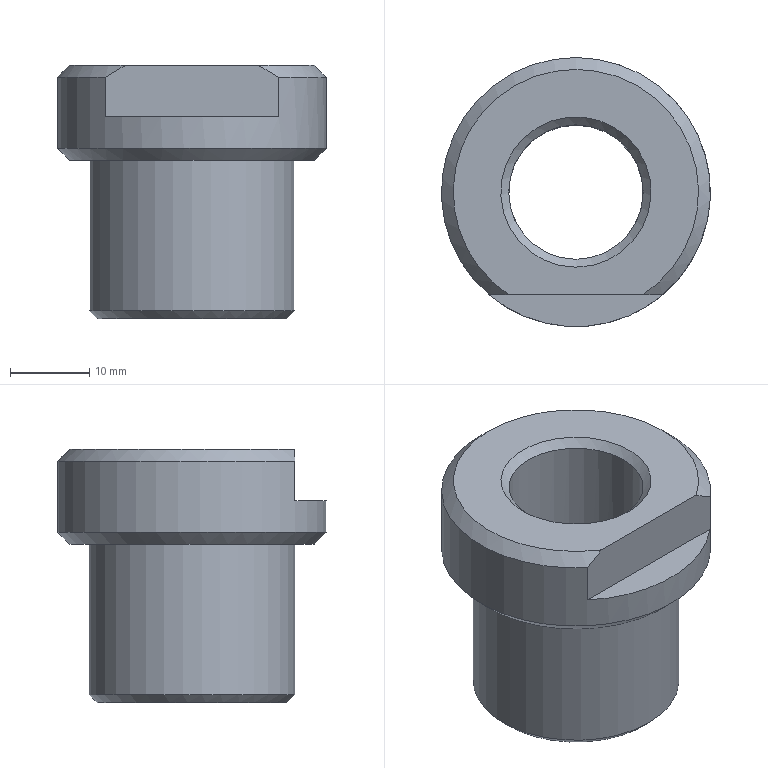Component | NX | DRILL_BUSH_4 | 1 solid | 13 faces | box 34 x 34 x 32 mm | volume 13557 mm3 | plane 5 | cone 5 | cylinder 3 | commonest cylinder face diameters 26 x1 34 x1 17 x1
STEP:
#1=CARTESIAN_POINT('',(0.,0.,0.));
#2=DIRECTION('',(0.,0.,1.));
#3=DIRECTION('',(1.,0.,0.));
#4=AXIS2_PLACEMENT_3D('',#1,#2,#3);
#5=CARTESIAN_POINT('',(62.5,-55.5,100.));
#6=VERTEX_POINT('',#5);
#7=CARTESIAN_POINT('',(62.5,-65.,100.));
#8=DIRECTION('',(0.,0.,1.));
#9=DIRECTION('',(0.,1.,0.));
#10=AXIS2_PLACEMENT_3D('',#7,#8,#9);
#11=CIRCLE('',#10,9.5);
#12=CARTESIAN_POINT('',(62.5,-65.,100.));
#13=DIRECTION('',(0.,0.,-1.));
#14=DIRECTION('',(0.,1.,0.));
#15=AXIS2_PLACEMENT_3D('',#12,#13,#14);
#16=PLANE('',#15);
#17=CARTESIAN_POINT('',(9.5,0.));
#18=CARTESIAN_POINT('',(9.5,-16.454));
#19=CARTESIAN_POINT('',(-4.75,-8.227));
#20=CARTESIAN_POINT('',(-19.,-0.));
#21=CARTESIAN_POINT('',(-4.75,8.227));
#22=CARTESIAN_POINT('',(9.5,16.454));
#23=CARTESIAN_POINT('',(9.5,0.));
#24=(BOUNDED_CURVE()B_SPLINE_CURVE(2,(#17,#18,#19,#20,#21,#22,#23),.UNSPECIFIED.,.T.,.F.)B_SPLINE_CURVE_WITH_KNOTS((1,2,2,2,2,1),(-2.094,0.,2.094,4.189,6.283,8.378),.UNSPECIFIED.)CURVE()GEOMETRIC_REPRESENTATION_ITEM()RATIONAL_B_SPLINE_CURVE((1.,0.5,1.,0.5,1.,0.5,1.))REPRESENTATION_ITEM(''));
#25=(GEOMETRIC_REPRESENTATION_CONTEXT(2)PARAMETRIC_REPRESENTATION_CONTEXT()REPRESENTATION_CONTEXT('',''));
#26=DEFINITIONAL_REPRESENTATION('',(#24),#25);
#27=PCURVE('',#16,#26);
#28=CARTESIAN_POINT('',(62.5,-65.,101.));
#29=DIRECTION('',(0.,0.,-1.));
#30=DIRECTION('',(0.,1.,0.));
#31=AXIS2_PLACEMENT_3D('',#28,#29,#30);
#32=CONICAL_SURFACE('',#31,8.5,0.7854);
#33=CARTESIAN_POINT('',(6.283,1.));
#34=DIRECTION('',(-1.,0.));
#35=VECTOR('',#34,1.);
#36=LINE('',#33,#35);
#37=(GEOMETRIC_REPRESENTATION_CONTEXT(2)PARAMETRIC_REPRESENTATION_CONTEXT()REPRESENTATION_CONTEXT('',''));
#38=DEFINITIONAL_REPRESENTATION('',(#36),#37);
#39=PCURVE('',#32,#38);
#40=SURFACE_CURVE('',#11,(#27,#39),.PCURVE_S1.);
#41=EDGE_CURVE('',#6,#6,#40,.T.);
#42=ORIENTED_EDGE('',*,*,#41,.T.);
#43=EDGE_LOOP('',(#42));
#44=FACE_BOUND('',#43,.T.);
#45=CARTESIAN_POINT('',(62.5,-53.,100.));
#46=VERTEX_POINT('',#45);
#47=CARTESIAN_POINT('',(62.5,-65.,100.));
#48=DIRECTION('',(0.,0.,-1.));
#49=DIRECTION('',(0.,1.,0.));
#50=AXIS2_PLACEMENT_3D('',#47,#48,#49);
#51=CIRCLE('',#50,12.);
#52=CARTESIAN_POINT('',(0.,0.));
#53=DIRECTION('',(1.,0.));
#54=AXIS2_PLACEMENT_2D('',#52,#53);
#55=CIRCLE('',#54,12.);
#56=(GEOMETRIC_REPRESENTATION_CONTEXT(2)PARAMETRIC_REPRESENTATION_CONTEXT()REPRESENTATION_CONTEXT('',''));
#57=DEFINITIONAL_REPRESENTATION('',(#55),#56);
#58=PCURVE('',#16,#57);
#59=CARTESIAN_POINT('',(62.5,-65.,101.));
#60=DIRECTION('',(0.,0.,1.));
#61=DIRECTION('',(0.,-1.,0.));
#62=AXIS2_PLACEMENT_3D('',#59,#60,#61);
#63=CONICAL_SURFACE('',#62,13.,0.7854);
#64=CARTESIAN_POINT('',(9.425,-1.));
#65=DIRECTION('',(-1.,0.));
#66=VECTOR('',#65,1.);
#67=LINE('',#64,#66);
#68=(GEOMETRIC_REPRESENTATION_CONTEXT(2)PARAMETRIC_REPRESENTATION_CONTEXT()REPRESENTATION_CONTEXT('',''));
#69=DEFINITIONAL_REPRESENTATION('',(#67),#68);
#70=PCURVE('',#63,#69);
#71=SURFACE_CURVE('',#51,(#58,#70),.PCURVE_S1.);
#72=EDGE_CURVE('',#46,#46,#71,.T.);
#73=ORIENTED_EDGE('',*,*,#72,.T.);
#74=EDGE_LOOP('',(#73));
#75=FACE_BOUND('',#74,.T.);
#76=ADVANCED_FACE('',(#44,#75),#16,.T.);
#77=CARTESIAN_POINT('',(62.5,-52.,101.));
#78=VERTEX_POINT('',#77);
#79=CARTESIAN_POINT('',(62.5,-65.,101.));
#80=DIRECTION('',(0.,0.,1.));
#81=DIRECTION('',(0.,1.,0.));
#82=AXIS2_PLACEMENT_3D('',#79,#80,#81);
#83=CIRCLE('',#82,13.);
#84=CARTESIAN_POINT('',(62.5,-65.,100.));
#85=DIRECTION('',(0.,0.,1.));
#86=DIRECTION('',(0.,-1.,0.));
#87=AXIS2_PLACEMENT_3D('',#84,#85,#86);
#88=CYLINDRICAL_SURFACE('',#87,13.);
#89=CARTESIAN_POINT('',(3.142,1.));
#90=DIRECTION('',(1.,0.));
#91=VECTOR('',#90,1.);
#92=LINE('',#89,#91);
#93=(GEOMETRIC_REPRESENTATION_CONTEXT(2)PARAMETRIC_REPRESENTATION_CONTEXT()REPRESENTATION_CONTEXT('',''));
#94=DEFINITIONAL_REPRESENTATION('',(#92),#93);
#95=PCURVE('',#88,#94);
#96=CARTESIAN_POINT('',(3.142,0.));
#97=DIRECTION('',(1.,0.));
#98=VECTOR('',#97,1.);
#99=LINE('',#96,#98);
#100=(GEOMETRIC_REPRESENTATION_CONTEXT(2)PARAMETRIC_REPRESENTATION_CONTEXT()REPRESENTATION_CONTEXT('',''));
#101=DEFINITIONAL_REPRESENTATION('',(#99),#100);
#102=PCURVE('',#63,#101);
#103=SURFACE_CURVE('',#83,(#95,#102),.PCURVE_S1.);
#104=EDGE_CURVE('',#78,#78,#103,.T.);
#105=ORIENTED_EDGE('',*,*,#104,.T.);
#106=CARTESIAN_POINT('',(62.5,-52.,120.));
#107=VERTEX_POINT('',#106);
#108=CARTESIAN_POINT('',(62.5,-52.,101.));
#109=CARTESIAN_POINT('',(62.5,-52.,120.));
#110=B_SPLINE_CURVE_WITH_KNOTS('',1,(#108,#109),.UNSPECIFIED.,.F.,.F.,(2,2),(1.,20.),.PIECEWISE_BEZIER_KNOTS.);
#111=CARTESIAN_POINT('',(9.425,0.));
#112=DIRECTION('',(0.,1.));
#113=VECTOR('',#112,1.);
#114=LINE('',#111,#113);
#115=(GEOMETRIC_REPRESENTATION_CONTEXT(2)PARAMETRIC_REPRESENTATION_CONTEXT()REPRESENTATION_CONTEXT('',''));
#116=DEFINITIONAL_REPRESENTATION('',(#114),#115);
#117=PCURVE('',#88,#116);
#118=CARTESIAN_POINT('',(3.142,0.));
#119=DIRECTION('',(0.,1.));
#120=VECTOR('',#119,1.);
#121=LINE('',#118,#120);
#122=(GEOMETRIC_REPRESENTATION_CONTEXT(2)PARAMETRIC_REPRESENTATION_CONTEXT()REPRESENTATION_CONTEXT('',''));
#123=DEFINITIONAL_REPRESENTATION('',(#121),#122);
#124=PCURVE('',#88,#123);
#125=SEAM_CURVE('',#110,(#117,#124),.PCURVE_S1.);
#126=EDGE_CURVE('',#78,#107,#125,.T.);
#127=ORIENTED_EDGE('',*,*,#126,.T.);
#128=CARTESIAN_POINT('',(62.5,-65.,120.));
#129=DIRECTION('',(0.,0.,1.));
#130=DIRECTION('',(0.,1.,0.));
#131=AXIS2_PLACEMENT_3D('',#128,#129,#130);
#132=CIRCLE('',#131,13.);
#133=CARTESIAN_POINT('',(3.142,20.));
#134=DIRECTION('',(1.,0.));
#135=VECTOR('',#134,1.);
#136=LINE('',#133,#135);
#137=(GEOMETRIC_REPRESENTATION_CONTEXT(2)PARAMETRIC_REPRESENTATION_CONTEXT()REPRESENTATION_CONTEXT('',''));
#138=DEFINITIONAL_REPRESENTATION('',(#136),#137);
#139=PCURVE('',#88,#138);
#140=CARTESIAN_POINT('',(62.5,-65.,120.));
#141=DIRECTION('',(0.,0.,-1.));
#142=DIRECTION('',(0.,1.,0.));
#143=AXIS2_PLACEMENT_3D('',#140,#141,#142);
#144=PLANE('',#143);
#145=CARTESIAN_POINT('',(13.,0.));
#146=CARTESIAN_POINT('',(13.,-22.517));
#147=CARTESIAN_POINT('',(-6.5,-11.258));
#148=CARTESIAN_POINT('',(-26.,-0.));
#149=CARTESIAN_POINT('',(-6.5,11.258));
#150=CARTESIAN_POINT('',(13.,22.517));
#151=CARTESIAN_POINT('',(13.,0.));
#152=(BOUNDED_CURVE()B_SPLINE_CURVE(2,(#145,#146,#147,#148,#149,#150,#151),.UNSPECIFIED.,.T.,.F.)B_SPLINE_CURVE_WITH_KNOTS((1,2,2,2,2,1),(-2.094,0.,2.094,4.189,6.283,8.378),.UNSPECIFIED.)CURVE()GEOMETRIC_REPRESENTATION_ITEM()RATIONAL_B_SPLINE_CURVE((1.,0.5,1.,0.5,1.,0.5,1.))REPRESENTATION_ITEM(''));
#153=(GEOMETRIC_REPRESENTATION_CONTEXT(2)PARAMETRIC_REPRESENTATION_CONTEXT()REPRESENTATION_CONTEXT('',''));
#154=DEFINITIONAL_REPRESENTATION('',(#152),#153);
#155=PCURVE('',#144,#154);
#156=SURFACE_CURVE('',#132,(#139,#155),.PCURVE_S1.);
#157=EDGE_CURVE('',#107,#107,#156,.T.);
#158=ORIENTED_EDGE('',*,*,#157,.F.);
#159=ORIENTED_EDGE('',*,*,#126,.F.);
#160=EDGE_LOOP('',(#105,#127,#158,#159));
#161=FACE_BOUND('',#160,.T.);
#162=ADVANCED_FACE('',(#161),#88,.T.);
#163=CARTESIAN_POINT('',(62.5,-74.5,132.));
#164=VERTEX_POINT('',#163);
#165=CARTESIAN_POINT('',(62.5,-65.,132.));
#166=DIRECTION('',(0.,0.,-1.));
#167=DIRECTION('',(0.,-1.,0.));
#168=AXIS2_PLACEMENT_3D('',#165,#166,#167);
#169=CIRCLE('',#168,9.5);
#170=CARTESIAN_POINT('',(62.5,-65.,132.));
#171=DIRECTION('',(0.,0.,1.));
#172=DIRECTION('',(0.,-1.,0.));
#173=AXIS2_PLACEMENT_3D('',#170,#171,#172);
#174=PLANE('',#173);
#175=CARTESIAN_POINT('',(9.5,0.));
#176=CARTESIAN_POINT('',(9.5,-16.454));
#177=CARTESIAN_POINT('',(-4.75,-8.227));
#178=CARTESIAN_POINT('',(-19.,-0.));
#179=CARTESIAN_POINT('',(-4.75,8.227));
#180=CARTESIAN_POINT('',(9.5,16.454));
#181=CARTESIAN_POINT('',(9.5,0.));
#182=(BOUNDED_CURVE()B_SPLINE_CURVE(2,(#175,#176,#177,#178,#179,#180,#181),.UNSPECIFIED.,.T.,.F.)B_SPLINE_CURVE_WITH_KNOTS((1,2,2,2,2,1),(-2.094,0.,2.094,4.189,6.283,8.378),.UNSPECIFIED.)CURVE()GEOMETRIC_REPRESENTATION_ITEM()RATIONAL_B_SPLINE_CURVE((1.,0.5,1.,0.5,1.,0.5,1.))REPRESENTATION_ITEM(''));
#183=(GEOMETRIC_REPRESENTATION_CONTEXT(2)PARAMETRIC_REPRESENTATION_CONTEXT()REPRESENTATION_CONTEXT('',''));
#184=DEFINITIONAL_REPRESENTATION('',(#182),#183);
#185=PCURVE('',#174,#184);
#186=CARTESIAN_POINT('',(62.5,-65.,132.));
#187=DIRECTION('',(0.,0.,1.));
#188=DIRECTION('',(0.,-1.,0.));
#189=AXIS2_PLACEMENT_3D('',#186,#187,#188);
#190=CONICAL_SURFACE('',#189,9.5,0.7854);
#191=CARTESIAN_POINT('',(6.283,0.));
#192=DIRECTION('',(-1.,0.));
#193=VECTOR('',#192,1.);
#194=LINE('',#191,#193);
#195=(GEOMETRIC_REPRESENTATION_CONTEXT(2)PARAMETRIC_REPRESENTATION_CONTEXT()REPRESENTATION_CONTEXT('',''));
#196=DEFINITIONAL_REPRESENTATION('',(#194),#195);
#197=PCURVE('',#190,#196);
#198=SURFACE_CURVE('',#169,(#185,#197),.PCURVE_S1.);
#199=EDGE_CURVE('',#164,#164,#198,.T.);
#200=ORIENTED_EDGE('',*,*,#199,.T.);
#201=EDGE_LOOP('',(#200));
#202=FACE_BOUND('',#201,.T.);
#203=CARTESIAN_POINT('',(70.941,-78.,132.));
#204=VERTEX_POINT('',#203);
#205=CARTESIAN_POINT('',(54.059,-78.,132.));
#206=VERTEX_POINT('',#205);
#207=CARTESIAN_POINT('',(84.5,-78.,132.));
#208=DIRECTION('',(-1.,-0.,0.));
#209=VECTOR('',#208,1.);
#210=LINE('',#207,#209);
#211=CARTESIAN_POINT('',(13.,22.));
#212=DIRECTION('',(0.,-1.));
#213=VECTOR('',#212,1.);
#214=LINE('',#211,#213);
#215=(GEOMETRIC_REPRESENTATION_CONTEXT(2)PARAMETRIC_REPRESENTATION_CONTEXT()REPRESENTATION_CONTEXT('',''));
#216=DEFINITIONAL_REPRESENTATION('',(#214),#215);
#217=PCURVE('',#174,#216);
#218=CARTESIAN_POINT('',(84.5,-78.,125.5));
#219=DIRECTION('',(-0.,1.,0.));
#220=DIRECTION('',(-1.,-0.,0.));
#221=AXIS2_PLACEMENT_3D('',#218,#219,#220);
#222=PLANE('',#221);
#223=CARTESIAN_POINT('',(0.,6.5));
#224=DIRECTION('',(1.,0.));
#225=VECTOR('',#224,1.);
#226=LINE('',#223,#225);
#227=(GEOMETRIC_REPRESENTATION_CONTEXT(2)PARAMETRIC_REPRESENTATION_CONTEXT()REPRESENTATION_CONTEXT('',''));
#228=DEFINITIONAL_REPRESENTATION('',(#226),#227);
#229=PCURVE('',#222,#228);
#230=SURFACE_CURVE('',#210,(#217,#229),.PCURVE_S1.);
#231=EDGE_CURVE('',#204,#206,#230,.T.);
#232=ORIENTED_EDGE('',*,*,#231,.F.);
#233=CARTESIAN_POINT('',(62.5,-65.,132.));
#234=DIRECTION('',(0.,0.,1.));
#235=DIRECTION('',(0.,-1.,0.));
#236=AXIS2_PLACEMENT_3D('',#233,#234,#235);
#237=CIRCLE('',#236,15.5);
#238=CARTESIAN_POINT('',(0.,0.));
#239=DIRECTION('',(1.,0.));
#240=AXIS2_PLACEMENT_2D('',#238,#239);
#241=CIRCLE('',#240,15.5);
#242=(GEOMETRIC_REPRESENTATION_CONTEXT(2)PARAMETRIC_REPRESENTATION_CONTEXT()REPRESENTATION_CONTEXT('',''));
#243=DEFINITIONAL_REPRESENTATION('',(#241),#242);
#244=PCURVE('',#174,#243);
#245=CARTESIAN_POINT('',(62.5,-65.,130.5));
#246=DIRECTION('',(0.,0.,-1.));
#247=DIRECTION('',(0.,1.,0.));
#248=AXIS2_PLACEMENT_3D('',#245,#246,#247);
#249=CONICAL_SURFACE('',#248,17.,0.7854);
#250=CARTESIAN_POINT('',(9.425,-1.5));
#251=DIRECTION('',(-1.,-0.));
#252=VECTOR('',#251,1.);
#253=LINE('',#250,#252);
#254=(GEOMETRIC_REPRESENTATION_CONTEXT(2)PARAMETRIC_REPRESENTATION_CONTEXT()REPRESENTATION_CONTEXT('',''));
#255=DEFINITIONAL_REPRESENTATION('',(#253),#254);
#256=PCURVE('',#249,#255);
#257=SURFACE_CURVE('',#237,(#244,#256),.PCURVE_S1.);
#258=EDGE_CURVE('',#204,#206,#257,.T.);
#259=ORIENTED_EDGE('',*,*,#258,.T.);
#260=EDGE_LOOP('',(#232,#259));
#261=FACE_BOUND('',#260,.T.);
#262=ADVANCED_FACE('',(#202,#261),#174,.T.);
#263=CARTESIAN_POINT('',(62.5,-49.5,120.));
#264=VERTEX_POINT('',#263);
#265=CARTESIAN_POINT('',(62.5,-65.,120.));
#266=DIRECTION('',(0.,0.,-1.));
#267=DIRECTION('',(0.,1.,0.));
#268=AXIS2_PLACEMENT_3D('',#265,#266,#267);
#269=CIRCLE('',#268,15.5);
#270=CARTESIAN_POINT('',(0.,0.));
#271=DIRECTION('',(1.,0.));
#272=AXIS2_PLACEMENT_2D('',#270,#271);
#273=CIRCLE('',#272,15.5);
#274=(GEOMETRIC_REPRESENTATION_CONTEXT(2)PARAMETRIC_REPRESENTATION_CONTEXT()REPRESENTATION_CONTEXT('',''));
#275=DEFINITIONAL_REPRESENTATION('',(#273),#274);
#276=PCURVE('',#144,#275);
#277=CARTESIAN_POINT('',(62.5,-65.,121.5));
#278=DIRECTION('',(0.,0.,1.));
#279=DIRECTION('',(0.,-1.,0.));
#280=AXIS2_PLACEMENT_3D('',#277,#278,#279);
#281=CONICAL_SURFACE('',#280,17.,0.7854);
#282=CARTESIAN_POINT('',(9.425,-1.5));
#283=DIRECTION('',(-1.,0.));
#284=VECTOR('',#283,1.);
#285=LINE('',#282,#284);
#286=(GEOMETRIC_REPRESENTATION_CONTEXT(2)PARAMETRIC_REPRESENTATION_CONTEXT()REPRESENTATION_CONTEXT('',''));
#287=DEFINITIONAL_REPRESENTATION('',(#285),#286);
#288=PCURVE('',#281,#287);
#289=SURFACE_CURVE('',#269,(#276,#288),.PCURVE_S1.);
#290=EDGE_CURVE('',#264,#264,#289,.T.);
#291=ORIENTED_EDGE('',*,*,#290,.T.);
#292=EDGE_LOOP('',(#291));
#293=FACE_BOUND('',#292,.T.);
#294=ORIENTED_EDGE('',*,*,#157,.T.);
#295=EDGE_LOOP('',(#294));
#296=FACE_BOUND('',#295,.T.);
#297=ADVANCED_FACE('',(#293,#296),#144,.T.);
#298=CARTESIAN_POINT('',(62.5,-48.,121.5));
#299=VERTEX_POINT('',#298);
#300=CARTESIAN_POINT('',(51.546,-78.,121.5));
#301=VERTEX_POINT('',#300);
#302=CARTESIAN_POINT('',(62.5,-65.,121.5));
#303=DIRECTION('',(0.,0.,1.));
#304=DIRECTION('',(0.,1.,0.));
#305=AXIS2_PLACEMENT_3D('',#302,#303,#304);
#306=CIRCLE('',#305,17.);
#307=CARTESIAN_POINT('',(62.5,-65.,120.));
#308=DIRECTION('',(0.,0.,1.));
#309=DIRECTION('',(0.,-1.,0.));
#310=AXIS2_PLACEMENT_3D('',#307,#308,#309);
#311=CYLINDRICAL_SURFACE('',#310,17.);
#312=CARTESIAN_POINT('',(9.425,1.5));
#313=DIRECTION('',(1.,0.));
#314=VECTOR('',#313,1.);
#315=LINE('',#312,#314);
#316=(GEOMETRIC_REPRESENTATION_CONTEXT(2)PARAMETRIC_REPRESENTATION_CONTEXT()REPRESENTATION_CONTEXT('',''));
#317=DEFINITIONAL_REPRESENTATION('',(#315),#316);
#318=PCURVE('',#311,#317);
#319=CARTESIAN_POINT('',(3.142,0.));
#320=DIRECTION('',(1.,0.));
#321=VECTOR('',#320,1.);
#322=LINE('',#319,#321);
#323=(GEOMETRIC_REPRESENTATION_CONTEXT(2)PARAMETRIC_REPRESENTATION_CONTEXT()REPRESENTATION_CONTEXT('',''));
#324=DEFINITIONAL_REPRESENTATION('',(#322),#323);
#325=PCURVE('',#281,#324);
#326=SURFACE_CURVE('',#306,(#318,#325),.PCURVE_S1.);
#327=EDGE_CURVE('',#299,#301,#326,.T.);
#328=ORIENTED_EDGE('',*,*,#327,.T.);
#329=CARTESIAN_POINT('',(51.546,-78.,125.5));
#330=VERTEX_POINT('',#329);
#331=CARTESIAN_POINT('',(51.546,-78.,121.5));
#332=CARTESIAN_POINT('',(51.546,-78.,125.5));
#333=B_SPLINE_CURVE_WITH_KNOTS('',1,(#331,#332),.UNSPECIFIED.,.F.,.F.,(2,2),(1.5,5.5),.PIECEWISE_BEZIER_KNOTS.);
#334=CARTESIAN_POINT('',(11.866,0.));
#335=DIRECTION('',(0.,1.));
#336=VECTOR('',#335,1.);
#337=LINE('',#334,#336);
#338=(GEOMETRIC_REPRESENTATION_CONTEXT(2)PARAMETRIC_REPRESENTATION_CONTEXT()REPRESENTATION_CONTEXT('',''));
#339=DEFINITIONAL_REPRESENTATION('',(#337),#338);
#340=PCURVE('',#311,#339);
#341=CARTESIAN_POINT('',(5.583,0.));
#342=DIRECTION('',(0.,1.));
#343=VECTOR('',#342,1.);
#344=LINE('',#341,#343);
#345=(GEOMETRIC_REPRESENTATION_CONTEXT(2)PARAMETRIC_REPRESENTATION_CONTEXT()REPRESENTATION_CONTEXT('',''));
#346=DEFINITIONAL_REPRESENTATION('',(#344),#345);
#347=PCURVE('',#311,#346);
#348=SEAM_CURVE('',#333,(#340,#347),.PCURVE_S1.);
#349=EDGE_CURVE('',#301,#330,#348,.T.);
#350=ORIENTED_EDGE('',*,*,#349,.T.);
#351=CARTESIAN_POINT('',(51.546,-78.,130.5));
#352=VERTEX_POINT('',#351);
#353=CARTESIAN_POINT('',(51.546,-78.,120.));
#354=DIRECTION('',(0.,0.,-1.));
#355=VECTOR('',#354,1.);
#356=LINE('',#353,#355);
#357=CARTESIAN_POINT('',(11.866,0.));
#358=DIRECTION('',(0.,-1.));
#359=VECTOR('',#358,1.);
#360=LINE('',#357,#359);
#361=(GEOMETRIC_REPRESENTATION_CONTEXT(2)PARAMETRIC_REPRESENTATION_CONTEXT()REPRESENTATION_CONTEXT('',''));
#362=DEFINITIONAL_REPRESENTATION('',(#360),#361);
#363=PCURVE('',#311,#362);
#364=CARTESIAN_POINT('',(32.954,-5.5));
#365=DIRECTION('',(0.,-1.));
#366=VECTOR('',#365,1.);
#367=LINE('',#364,#366);
#368=(GEOMETRIC_REPRESENTATION_CONTEXT(2)PARAMETRIC_REPRESENTATION_CONTEXT()REPRESENTATION_CONTEXT('',''));
#369=DEFINITIONAL_REPRESENTATION('',(#367),#368);
#370=PCURVE('',#222,#369);
#371=SURFACE_CURVE('',#356,(#363,#370),.PCURVE_S1.);
#372=EDGE_CURVE('',#352,#330,#371,.T.);
#373=ORIENTED_EDGE('',*,*,#372,.F.);
#374=CARTESIAN_POINT('',(73.454,-78.,130.5));
#375=VERTEX_POINT('',#374);
#376=CARTESIAN_POINT('',(62.5,-65.,130.5));
#377=DIRECTION('',(0.,0.,-1.));
#378=DIRECTION('',(0.,-1.,0.));
#379=AXIS2_PLACEMENT_3D('',#376,#377,#378);
#380=CIRCLE('',#379,17.);
#381=CARTESIAN_POINT('',(12.566,10.5));
#382=DIRECTION('',(-1.,0.));
#383=VECTOR('',#382,1.);
#384=LINE('',#381,#383);
#385=(GEOMETRIC_REPRESENTATION_CONTEXT(2)PARAMETRIC_REPRESENTATION_CONTEXT()REPRESENTATION_CONTEXT('',''));
#386=DEFINITIONAL_REPRESENTATION('',(#384),#385);
#387=PCURVE('',#311,#386);
#388=CARTESIAN_POINT('',(3.142,0.));
#389=DIRECTION('',(1.,-0.));
#390=VECTOR('',#389,1.);
#391=LINE('',#388,#390);
#392=(GEOMETRIC_REPRESENTATION_CONTEXT(2)PARAMETRIC_REPRESENTATION_CONTEXT()REPRESENTATION_CONTEXT('',''));
#393=DEFINITIONAL_REPRESENTATION('',(#391),#392);
#394=PCURVE('',#249,#393);
#395=SURFACE_CURVE('',#380,(#387,#394),.PCURVE_S1.);
#396=EDGE_CURVE('',#352,#375,#395,.T.);
#397=ORIENTED_EDGE('',*,*,#396,.T.);
#398=CARTESIAN_POINT('',(73.454,-78.,125.5));
#399=VERTEX_POINT('',#398);
#400=CARTESIAN_POINT('',(73.454,-78.,120.));
#401=DIRECTION('',(0.,0.,1.));
#402=VECTOR('',#401,1.);
#403=LINE('',#400,#402);
#404=CARTESIAN_POINT('',(6.983,0.));
#405=DIRECTION('',(0.,1.));
#406=VECTOR('',#405,1.);
#407=LINE('',#404,#406);
#408=(GEOMETRIC_REPRESENTATION_CONTEXT(2)PARAMETRIC_REPRESENTATION_CONTEXT()REPRESENTATION_CONTEXT('',''));
#409=DEFINITIONAL_REPRESENTATION('',(#407),#408);
#410=PCURVE('',#311,#409);
#411=CARTESIAN_POINT('',(11.046,-5.5));
#412=DIRECTION('',(0.,1.));
#413=VECTOR('',#412,1.);
#414=LINE('',#411,#413);
#415=(GEOMETRIC_REPRESENTATION_CONTEXT(2)PARAMETRIC_REPRESENTATION_CONTEXT()REPRESENTATION_CONTEXT('',''));
#416=DEFINITIONAL_REPRESENTATION('',(#414),#415);
#417=PCURVE('',#222,#416);
#418=SURFACE_CURVE('',#403,(#410,#417),.PCURVE_S1.);
#419=EDGE_CURVE('',#399,#375,#418,.T.);
#420=ORIENTED_EDGE('',*,*,#419,.F.);
#421=CARTESIAN_POINT('',(62.5,-65.,125.5));
#422=DIRECTION('',(0.,0.,-1.));
#423=DIRECTION('',(0.,-1.,0.));
#424=AXIS2_PLACEMENT_3D('',#421,#422,#423);
#425=CIRCLE('',#424,17.);
#426=CARTESIAN_POINT('',(12.566,5.5));
#427=DIRECTION('',(-1.,0.));
#428=VECTOR('',#427,1.);
#429=LINE('',#426,#428);
#430=(GEOMETRIC_REPRESENTATION_CONTEXT(2)PARAMETRIC_REPRESENTATION_CONTEXT()REPRESENTATION_CONTEXT('',''));
#431=DEFINITIONAL_REPRESENTATION('',(#429),#430);
#432=PCURVE('',#311,#431);
#433=CARTESIAN_POINT('',(62.5,-65.,125.5));
#434=DIRECTION('',(0.,0.,1.));
#435=DIRECTION('',(0.,-1.,0.));
#436=AXIS2_PLACEMENT_3D('',#433,#434,#435);
#437=PLANE('',#436);
#438=CARTESIAN_POINT('',(17.,0.));
#439=CARTESIAN_POINT('',(17.,-29.445));
#440=CARTESIAN_POINT('',(-8.5,-14.722));
#441=CARTESIAN_POINT('',(-34.,-0.));
#442=CARTESIAN_POINT('',(-8.5,14.722));
#443=CARTESIAN_POINT('',(17.,29.445));
#444=CARTESIAN_POINT('',(17.,0.));
#445=(BOUNDED_CURVE()B_SPLINE_CURVE(2,(#438,#439,#440,#441,#442,#443,#444),.UNSPECIFIED.,.T.,.F.)B_SPLINE_CURVE_WITH_KNOTS((1,2,2,2,2,1),(-2.094,0.,2.094,4.189,6.283,8.378),.UNSPECIFIED.)CURVE()GEOMETRIC_REPRESENTATION_ITEM()RATIONAL_B_SPLINE_CURVE((1.,0.5,1.,0.5,1.,0.5,1.))REPRESENTATION_ITEM(''));
#446=(GEOMETRIC_REPRESENTATION_CONTEXT(2)PARAMETRIC_REPRESENTATION_CONTEXT()REPRESENTATION_CONTEXT('',''));
#447=DEFINITIONAL_REPRESENTATION('',(#445),#446);
#448=PCURVE('',#437,#447);
#449=SURFACE_CURVE('',#425,(#432,#448),.PCURVE_S1.);
#450=EDGE_CURVE('',#399,#330,#449,.T.);
#451=ORIENTED_EDGE('',*,*,#450,.T.);
#452=ORIENTED_EDGE('',*,*,#349,.F.);
#453=CARTESIAN_POINT('',(62.5,-65.,121.5));
#454=DIRECTION('',(0.,0.,1.));
#455=DIRECTION('',(0.,1.,0.));
#456=AXIS2_PLACEMENT_3D('',#453,#454,#455);
#457=CIRCLE('',#456,17.);
#458=CARTESIAN_POINT('',(3.142,1.5));
#459=DIRECTION('',(1.,0.));
#460=VECTOR('',#459,1.);
#461=LINE('',#458,#460);
#462=(GEOMETRIC_REPRESENTATION_CONTEXT(2)PARAMETRIC_REPRESENTATION_CONTEXT()REPRESENTATION_CONTEXT('',''));
#463=DEFINITIONAL_REPRESENTATION('',(#461),#462);
#464=PCURVE('',#311,#463);
#465=CARTESIAN_POINT('',(3.142,0.));
#466=DIRECTION('',(1.,-0.));
#467=VECTOR('',#466,1.);
#468=LINE('',#465,#467);
#469=(GEOMETRIC_REPRESENTATION_CONTEXT(2)PARAMETRIC_REPRESENTATION_CONTEXT()REPRESENTATION_CONTEXT('',''));
#470=DEFINITIONAL_REPRESENTATION('',(#468),#469);
#471=PCURVE('',#281,#470);
#472=SURFACE_CURVE('',#457,(#464,#471),.PCURVE_S1.);
#473=EDGE_CURVE('',#301,#299,#472,.T.);
#474=ORIENTED_EDGE('',*,*,#473,.T.);
#475=EDGE_LOOP('',(#328,#350,#373,#397,#420,#451,#452,#474));
#476=FACE_BOUND('',#475,.T.);
#477=ADVANCED_FACE('',(#476),#311,.T.);
#478=CARTESIAN_POINT('',(62.5,-56.5,101.));
#479=VERTEX_POINT('',#478);
#480=CARTESIAN_POINT('',(62.5,-65.,101.));
#481=DIRECTION('',(0.,0.,-1.));
#482=DIRECTION('',(0.,1.,0.));
#483=AXIS2_PLACEMENT_3D('',#480,#481,#482);
#484=CIRCLE('',#483,8.5);
#485=CARTESIAN_POINT('',(62.5,-65.,132.));
#486=DIRECTION('',(0.,0.,-1.));
#487=DIRECTION('',(0.,1.,0.));
#488=AXIS2_PLACEMENT_3D('',#485,#486,#487);
#489=CYLINDRICAL_SURFACE('',#488,8.5);
#490=CARTESIAN_POINT('',(0.,31.));
#491=DIRECTION('',(1.,0.));
#492=VECTOR('',#491,1.);
#493=LINE('',#490,#492);
#494=(GEOMETRIC_REPRESENTATION_CONTEXT(2)PARAMETRIC_REPRESENTATION_CONTEXT()REPRESENTATION_CONTEXT('',''));
#495=DEFINITIONAL_REPRESENTATION('',(#493),#494);
#496=PCURVE('',#489,#495);
#497=CARTESIAN_POINT('',(0.,0.));
#498=DIRECTION('',(1.,0.));
#499=VECTOR('',#498,1.);
#500=LINE('',#497,#499);
#501=(GEOMETRIC_REPRESENTATION_CONTEXT(2)PARAMETRIC_REPRESENTATION_CONTEXT()REPRESENTATION_CONTEXT('',''));
#502=DEFINITIONAL_REPRESENTATION('',(#500),#501);
#503=PCURVE('',#32,#502);
#504=SURFACE_CURVE('',#484,(#496,#503),.PCURVE_S1.);
#505=EDGE_CURVE('',#479,#479,#504,.T.);
#506=ORIENTED_EDGE('',*,*,#505,.F.);
#507=CARTESIAN_POINT('',(62.5,-56.5,131.));
#508=VERTEX_POINT('',#507);
#509=CARTESIAN_POINT('',(62.5,-56.5,131.));
#510=CARTESIAN_POINT('',(62.5,-56.5,101.));
#511=B_SPLINE_CURVE_WITH_KNOTS('',1,(#509,#510),.UNSPECIFIED.,.F.,.F.,(2,2),(1.,31.),.PIECEWISE_BEZIER_KNOTS.);
#512=CARTESIAN_POINT('',(0.,0.));
#513=DIRECTION('',(0.,1.));
#514=VECTOR('',#513,1.);
#515=LINE('',#512,#514);
#516=(GEOMETRIC_REPRESENTATION_CONTEXT(2)PARAMETRIC_REPRESENTATION_CONTEXT()REPRESENTATION_CONTEXT('',''));
#517=DEFINITIONAL_REPRESENTATION('',(#515),#516);
#518=PCURVE('',#489,#517);
#519=CARTESIAN_POINT('',(6.283,0.));
#520=DIRECTION('',(0.,1.));
#521=VECTOR('',#520,1.);
#522=LINE('',#519,#521);
#523=(GEOMETRIC_REPRESENTATION_CONTEXT(2)PARAMETRIC_REPRESENTATION_CONTEXT()REPRESENTATION_CONTEXT('',''));
#524=DEFINITIONAL_REPRESENTATION('',(#522),#523);
#525=PCURVE('',#489,#524);
#526=SEAM_CURVE('',#511,(#518,#525),.PCURVE_S1.);
#527=EDGE_CURVE('',#508,#479,#526,.T.);
#528=ORIENTED_EDGE('',*,*,#527,.F.);
#529=CARTESIAN_POINT('',(62.5,-73.5,131.));
#530=VERTEX_POINT('',#529);
#531=CARTESIAN_POINT('',(62.5,-65.,131.));
#532=DIRECTION('',(0.,0.,1.));
#533=DIRECTION('',(0.,-1.,0.));
#534=AXIS2_PLACEMENT_3D('',#531,#532,#533);
#535=CIRCLE('',#534,8.5);
#536=CARTESIAN_POINT('',(3.142,1.));
#537=DIRECTION('',(-1.,0.));
#538=VECTOR('',#537,1.);
#539=LINE('',#536,#538);
#540=(GEOMETRIC_REPRESENTATION_CONTEXT(2)PARAMETRIC_REPRESENTATION_CONTEXT()REPRESENTATION_CONTEXT('',''));
#541=DEFINITIONAL_REPRESENTATION('',(#539),#540);
#542=PCURVE('',#489,#541);
#543=CARTESIAN_POINT('',(0.,-1.));
#544=DIRECTION('',(1.,0.));
#545=VECTOR('',#544,1.);
#546=LINE('',#543,#545);
#547=(GEOMETRIC_REPRESENTATION_CONTEXT(2)PARAMETRIC_REPRESENTATION_CONTEXT()REPRESENTATION_CONTEXT('',''));
#548=DEFINITIONAL_REPRESENTATION('',(#546),#547);
#549=PCURVE('',#190,#548);
#550=SURFACE_CURVE('',#535,(#542,#549),.PCURVE_S1.);
#551=EDGE_CURVE('',#530,#508,#550,.T.);
#552=ORIENTED_EDGE('',*,*,#551,.F.);
#553=CARTESIAN_POINT('',(62.5,-65.,131.));
#554=DIRECTION('',(0.,0.,1.));
#555=DIRECTION('',(0.,-1.,0.));
#556=AXIS2_PLACEMENT_3D('',#553,#554,#555);
#557=CIRCLE('',#556,8.5);
#558=CARTESIAN_POINT('',(9.425,1.));
#559=DIRECTION('',(-1.,0.));
#560=VECTOR('',#559,1.);
#561=LINE('',#558,#560);
#562=(GEOMETRIC_REPRESENTATION_CONTEXT(2)PARAMETRIC_REPRESENTATION_CONTEXT()REPRESENTATION_CONTEXT('',''));
#563=DEFINITIONAL_REPRESENTATION('',(#561),#562);
#564=PCURVE('',#489,#563);
#565=CARTESIAN_POINT('',(0.,-1.));
#566=DIRECTION('',(1.,0.));
#567=VECTOR('',#566,1.);
#568=LINE('',#565,#567);
#569=(GEOMETRIC_REPRESENTATION_CONTEXT(2)PARAMETRIC_REPRESENTATION_CONTEXT()REPRESENTATION_CONTEXT('',''));
#570=DEFINITIONAL_REPRESENTATION('',(#568),#569);
#571=PCURVE('',#190,#570);
#572=SURFACE_CURVE('',#557,(#564,#571),.PCURVE_S1.);
#573=EDGE_CURVE('',#508,#530,#572,.T.);
#574=ORIENTED_EDGE('',*,*,#573,.F.);
#575=ORIENTED_EDGE('',*,*,#527,.T.);
#576=EDGE_LOOP('',(#506,#528,#552,#574,#575));
#577=FACE_BOUND('',#576,.F.);
#578=ADVANCED_FACE('',(#577),#489,.F.);
#579=ORIENTED_EDGE('',*,*,#419,.T.);
#580=CARTESIAN_POINT('',(73.454,-78.,130.5));
#581=CARTESIAN_POINT('',(72.634,-78.,131.028));
#582=CARTESIAN_POINT('',(71.798,-78.,131.533));
#583=CARTESIAN_POINT('',(70.941,-78.,132.));
#584=B_SPLINE_CURVE_WITH_KNOTS('',3,(#580,#581,#582,#583),.UNSPECIFIED.,.F.,.F.,(4,4),(0.,1.),.PIECEWISE_BEZIER_KNOTS.);
#585=CARTESIAN_POINT('',(11.046,5.));
#586=CARTESIAN_POINT('',(11.866,5.528));
#587=CARTESIAN_POINT('',(12.702,6.033));
#588=CARTESIAN_POINT('',(13.559,6.5));
#589=B_SPLINE_CURVE_WITH_KNOTS('',3,(#585,#586,#587,#588),.UNSPECIFIED.,.F.,.F.,(4,4),(0.,1.),.PIECEWISE_BEZIER_KNOTS.);
#590=(GEOMETRIC_REPRESENTATION_CONTEXT(2)PARAMETRIC_REPRESENTATION_CONTEXT()REPRESENTATION_CONTEXT('',''));
#591=DEFINITIONAL_REPRESENTATION('',(#589),#590);
#592=PCURVE('',#222,#591);
#593=CARTESIAN_POINT('',(8.725,0.));
#594=CARTESIAN_POINT('',(8.726,-0.02402));
#595=CARTESIAN_POINT('',(8.73,-0.07197));
#596=CARTESIAN_POINT('',(8.735,-0.1436));
#597=CARTESIAN_POINT('',(8.74,-0.2149));
#598=CARTESIAN_POINT('',(8.745,-0.2859));
#599=CARTESIAN_POINT('',(8.75,-0.3565));
#600=CARTESIAN_POINT('',(8.756,-0.4269));
#601=CARTESIAN_POINT('',(8.761,-0.4968));
#602=CARTESIAN_POINT('',(8.767,-0.5665));
#603=CARTESIAN_POINT('',(8.772,-0.6358));
#604=CARTESIAN_POINT('',(8.778,-0.7047));
#605=CARTESIAN_POINT('',(8.783,-0.7732));
#606=CARTESIAN_POINT('',(8.789,-0.8414));
#607=CARTESIAN_POINT('',(8.795,-0.9091));
#608=CARTESIAN_POINT('',(8.8,-0.9765));
#609=CARTESIAN_POINT('',(8.806,-1.043));
#610=CARTESIAN_POINT('',(8.812,-1.11));
#611=CARTESIAN_POINT('',(8.818,-1.176));
#612=CARTESIAN_POINT('',(8.824,-1.242));
#613=CARTESIAN_POINT('',(8.83,-1.307));
#614=CARTESIAN_POINT('',(8.836,-1.372));
#615=CARTESIAN_POINT('',(8.843,-1.436));
#616=CARTESIAN_POINT('',(8.847,-1.479));
#617=CARTESIAN_POINT('',(8.849,-1.5));
#618=B_SPLINE_CURVE_WITH_KNOTS('',3,(#593,#594,#595,#596,#597,#598,#599,#600,#601,#602,#603,#604,#605,#606,#607,#608,#609,#610,#611,#612,#613,#614,#615,#616,#617),.UNSPECIFIED.,.F.,.F.,(4,1,1,1,1,1,1,1,1,1,1,1,1,1,1,1,1,1,1,1,1,1,4),(0.,0.04545,0.09091,0.1364,0.1818,0.2273,0.2727,0.3182,0.3636,0.4091,0.4545,0.5,0.5455,0.5909,0.6364,0.6818,0.7273,0.7727,0.8182,0.8636,0.9091,0.9545,1.),.QUASI_UNIFORM_KNOTS.);
#619=(GEOMETRIC_REPRESENTATION_CONTEXT(2)PARAMETRIC_REPRESENTATION_CONTEXT()REPRESENTATION_CONTEXT('',''));
#620=DEFINITIONAL_REPRESENTATION('',(#618),#619);
#621=PCURVE('',#249,#620);
#622=SURFACE_CURVE('',#584,(#592,#621),.PCURVE_S1.);
#623=EDGE_CURVE('',#375,#204,#622,.T.);
#624=ORIENTED_EDGE('',*,*,#623,.T.);
#625=ORIENTED_EDGE('',*,*,#231,.T.);
#626=CARTESIAN_POINT('',(54.059,-78.,132.));
#627=CARTESIAN_POINT('',(53.202,-78.,131.533));
#628=CARTESIAN_POINT('',(52.366,-78.,131.028));
#629=CARTESIAN_POINT('',(51.546,-78.,130.5));
#630=B_SPLINE_CURVE_WITH_KNOTS('',3,(#626,#627,#628,#629),.UNSPECIFIED.,.F.,.F.,(4,4),(0.,1.),.PIECEWISE_BEZIER_KNOTS.);
#631=CARTESIAN_POINT('',(30.441,6.5));
#632=CARTESIAN_POINT('',(31.298,6.033));
#633=CARTESIAN_POINT('',(32.134,5.528));
#634=CARTESIAN_POINT('',(32.954,5.));
#635=B_SPLINE_CURVE_WITH_KNOTS('',3,(#631,#632,#633,#634),.UNSPECIFIED.,.F.,.F.,(4,4),(0.,1.),.PIECEWISE_BEZIER_KNOTS.);
#636=(GEOMETRIC_REPRESENTATION_CONTEXT(2)PARAMETRIC_REPRESENTATION_CONTEXT()REPRESENTATION_CONTEXT('',''));
#637=DEFINITIONAL_REPRESENTATION('',(#635),#636);
#638=PCURVE('',#222,#637);
#639=CARTESIAN_POINT('',(3.717,-1.5));
#640=CARTESIAN_POINT('',(3.72,-1.479));
#641=CARTESIAN_POINT('',(3.724,-1.436));
#642=CARTESIAN_POINT('',(3.73,-1.372));
#643=CARTESIAN_POINT('',(3.736,-1.307));
#644=CARTESIAN_POINT('',(3.742,-1.242));
#645=CARTESIAN_POINT('',(3.748,-1.176));
#646=CARTESIAN_POINT('',(3.754,-1.11));
#647=CARTESIAN_POINT('',(3.76,-1.043));
#648=CARTESIAN_POINT('',(3.766,-0.9765));
#649=CARTESIAN_POINT('',(3.772,-0.9091));
#650=CARTESIAN_POINT('',(3.778,-0.8414));
#651=CARTESIAN_POINT('',(3.783,-0.7732));
#652=CARTESIAN_POINT('',(3.789,-0.7047));
#653=CARTESIAN_POINT('',(3.794,-0.6358));
#654=CARTESIAN_POINT('',(3.8,-0.5665));
#655=CARTESIAN_POINT('',(3.805,-0.4968));
#656=CARTESIAN_POINT('',(3.811,-0.4269));
#657=CARTESIAN_POINT('',(3.816,-0.3565));
#658=CARTESIAN_POINT('',(3.821,-0.2859));
#659=CARTESIAN_POINT('',(3.826,-0.2149));
#660=CARTESIAN_POINT('',(3.832,-0.1436));
#661=CARTESIAN_POINT('',(3.837,-0.07197));
#662=CARTESIAN_POINT('',(3.84,-0.02402));
#663=CARTESIAN_POINT('',(3.842,-0.));
#664=B_SPLINE_CURVE_WITH_KNOTS('',3,(#639,#640,#641,#642,#643,#644,#645,#646,#647,#648,#649,#650,#651,#652,#653,#654,#655,#656,#657,#658,#659,#660,#661,#662,#663),.UNSPECIFIED.,.F.,.F.,(4,1,1,1,1,1,1,1,1,1,1,1,1,1,1,1,1,1,1,1,1,1,4),(0.,0.04545,0.09091,0.1364,0.1818,0.2273,0.2727,0.3182,0.3636,0.4091,0.4545,0.5,0.5455,0.5909,0.6364,0.6818,0.7273,0.7727,0.8182,0.8636,0.9091,0.9545,1.),.QUASI_UNIFORM_KNOTS.);
#665=(GEOMETRIC_REPRESENTATION_CONTEXT(2)PARAMETRIC_REPRESENTATION_CONTEXT()REPRESENTATION_CONTEXT('',''));
#666=DEFINITIONAL_REPRESENTATION('',(#664),#665);
#667=PCURVE('',#249,#666);
#668=SURFACE_CURVE('',#630,(#638,#667),.PCURVE_S1.);
#669=EDGE_CURVE('',#206,#352,#668,.T.);
#670=ORIENTED_EDGE('',*,*,#669,.T.);
#671=ORIENTED_EDGE('',*,*,#372,.T.);
#672=CARTESIAN_POINT('',(84.5,-78.,125.5));
#673=DIRECTION('',(1.,0.,0.));
#674=VECTOR('',#673,1.);
#675=LINE('',#672,#674);
#676=CARTESIAN_POINT('',(0.,0.));
#677=DIRECTION('',(-1.,0.));
#678=VECTOR('',#677,1.);
#679=LINE('',#676,#678);
#680=(GEOMETRIC_REPRESENTATION_CONTEXT(2)PARAMETRIC_REPRESENTATION_CONTEXT()REPRESENTATION_CONTEXT('',''));
#681=DEFINITIONAL_REPRESENTATION('',(#679),#680);
#682=PCURVE('',#222,#681);
#683=CARTESIAN_POINT('',(13.,22.));
#684=DIRECTION('',(-0.,1.));
#685=VECTOR('',#684,1.);
#686=LINE('',#683,#685);
#687=(GEOMETRIC_REPRESENTATION_CONTEXT(2)PARAMETRIC_REPRESENTATION_CONTEXT()REPRESENTATION_CONTEXT('',''));
#688=DEFINITIONAL_REPRESENTATION('',(#686),#687);
#689=PCURVE('',#437,#688);
#690=SURFACE_CURVE('',#675,(#682,#689),.PCURVE_S1.);
#691=EDGE_CURVE('',#330,#399,#690,.T.);
#692=ORIENTED_EDGE('',*,*,#691,.T.);
#693=EDGE_LOOP('',(#579,#624,#625,#670,#671,#692));
#694=FACE_BOUND('',#693,.T.);
#695=ADVANCED_FACE('',(#694),#222,.F.);
#696=ORIENTED_EDGE('',*,*,#691,.F.);
#697=ORIENTED_EDGE('',*,*,#450,.F.);
#698=EDGE_LOOP('',(#696,#697));
#699=FACE_BOUND('',#698,.T.);
#700=ADVANCED_FACE('',(#699),#437,.T.);
#701=ORIENTED_EDGE('',*,*,#290,.F.);
#702=CARTESIAN_POINT('',(62.5,-49.5,120.));
#703=CARTESIAN_POINT('',(62.5,-48.,121.5));
#704=B_SPLINE_CURVE_WITH_KNOTS('',1,(#702,#703),.UNSPECIFIED.,.F.,.F.,(2,2),(-2.121,0.),.PIECEWISE_BEZIER_KNOTS.);
#705=CARTESIAN_POINT('',(9.425,0.));
#706=DIRECTION('',(0.,1.));
#707=VECTOR('',#706,1.);
#708=LINE('',#705,#707);
#709=(GEOMETRIC_REPRESENTATION_CONTEXT(2)PARAMETRIC_REPRESENTATION_CONTEXT()REPRESENTATION_CONTEXT('',''));
#710=DEFINITIONAL_REPRESENTATION('',(#708),#709);
#711=PCURVE('',#281,#710);
#712=CARTESIAN_POINT('',(3.142,0.));
#713=DIRECTION('',(0.,1.));
#714=VECTOR('',#713,1.);
#715=LINE('',#712,#714);
#716=(GEOMETRIC_REPRESENTATION_CONTEXT(2)PARAMETRIC_REPRESENTATION_CONTEXT()REPRESENTATION_CONTEXT('',''));
#717=DEFINITIONAL_REPRESENTATION('',(#715),#716);
#718=PCURVE('',#281,#717);
#719=SEAM_CURVE('',#704,(#711,#718),.PCURVE_S1.);
#720=EDGE_CURVE('',#264,#299,#719,.T.);
#721=ORIENTED_EDGE('',*,*,#720,.T.);
#722=ORIENTED_EDGE('',*,*,#473,.F.);
#723=ORIENTED_EDGE('',*,*,#327,.F.);
#724=ORIENTED_EDGE('',*,*,#720,.F.);
#725=EDGE_LOOP('',(#701,#721,#722,#723,#724));
#726=FACE_BOUND('',#725,.T.);
#727=ADVANCED_FACE('',(#726),#281,.T.);
#728=ORIENTED_EDGE('',*,*,#669,.F.);
#729=ORIENTED_EDGE('',*,*,#258,.F.);
#730=ORIENTED_EDGE('',*,*,#623,.F.);
#731=ORIENTED_EDGE('',*,*,#396,.F.);
#732=EDGE_LOOP('',(#728,#729,#730,#731));
#733=FACE_BOUND('',#732,.T.);
#734=ADVANCED_FACE('',(#733),#249,.T.);
#735=ORIENTED_EDGE('',*,*,#41,.T.);
#736=CARTESIAN_POINT('',(62.5,-56.5,101.));
#737=CARTESIAN_POINT('',(62.5,-55.5,100.));
#738=B_SPLINE_CURVE_WITH_KNOTS('',1,(#736,#737),.UNSPECIFIED.,.F.,.F.,(2,2),(0.,1.414),.PIECEWISE_BEZIER_KNOTS.);
#739=CARTESIAN_POINT('',(0.,0.));
#740=DIRECTION('',(0.,1.));
#741=VECTOR('',#740,1.);
#742=LINE('',#739,#741);
#743=(GEOMETRIC_REPRESENTATION_CONTEXT(2)PARAMETRIC_REPRESENTATION_CONTEXT()REPRESENTATION_CONTEXT('',''));
#744=DEFINITIONAL_REPRESENTATION('',(#742),#743);
#745=PCURVE('',#32,#744);
#746=CARTESIAN_POINT('',(6.283,0.));
#747=DIRECTION('',(0.,1.));
#748=VECTOR('',#747,1.);
#749=LINE('',#746,#748);
#750=(GEOMETRIC_REPRESENTATION_CONTEXT(2)PARAMETRIC_REPRESENTATION_CONTEXT()REPRESENTATION_CONTEXT('',''));
#751=DEFINITIONAL_REPRESENTATION('',(#749),#750);
#752=PCURVE('',#32,#751);
#753=SEAM_CURVE('',#738,(#745,#752),.PCURVE_S1.);
#754=EDGE_CURVE('',#479,#6,#753,.T.);
#755=ORIENTED_EDGE('',*,*,#754,.F.);
#756=ORIENTED_EDGE('',*,*,#505,.T.);
#757=ORIENTED_EDGE('',*,*,#754,.T.);
#758=EDGE_LOOP('',(#735,#755,#756,#757));
#759=FACE_BOUND('',#758,.F.);
#760=ADVANCED_FACE('',(#759),#32,.F.);
#761=ORIENTED_EDGE('',*,*,#72,.F.);
#762=CARTESIAN_POINT('',(62.5,-53.,100.));
#763=CARTESIAN_POINT('',(62.5,-52.,101.));
#764=B_SPLINE_CURVE_WITH_KNOTS('',1,(#762,#763),.UNSPECIFIED.,.F.,.F.,(2,2),(-1.414,0.),.PIECEWISE_BEZIER_KNOTS.);
#765=CARTESIAN_POINT('',(9.425,0.));
#766=DIRECTION('',(0.,1.));
#767=VECTOR('',#766,1.);
#768=LINE('',#765,#767);
#769=(GEOMETRIC_REPRESENTATION_CONTEXT(2)PARAMETRIC_REPRESENTATION_CONTEXT()REPRESENTATION_CONTEXT('',''));
#770=DEFINITIONAL_REPRESENTATION('',(#768),#769);
#771=PCURVE('',#63,#770);
#772=CARTESIAN_POINT('',(3.142,0.));
#773=DIRECTION('',(0.,1.));
#774=VECTOR('',#773,1.);
#775=LINE('',#772,#774);
#776=(GEOMETRIC_REPRESENTATION_CONTEXT(2)PARAMETRIC_REPRESENTATION_CONTEXT()REPRESENTATION_CONTEXT('',''));
#777=DEFINITIONAL_REPRESENTATION('',(#775),#776);
#778=PCURVE('',#63,#777);
#779=SEAM_CURVE('',#764,(#771,#778),.PCURVE_S1.);
#780=EDGE_CURVE('',#46,#78,#779,.T.);
#781=ORIENTED_EDGE('',*,*,#780,.T.);
#782=ORIENTED_EDGE('',*,*,#104,.F.);
#783=ORIENTED_EDGE('',*,*,#780,.F.);
#784=EDGE_LOOP('',(#761,#781,#782,#783));
#785=FACE_BOUND('',#784,.T.);
#786=ADVANCED_FACE('',(#785),#63,.T.);
#787=ORIENTED_EDGE('',*,*,#573,.T.);
#788=CARTESIAN_POINT('',(62.5,-73.5,131.));
#789=CARTESIAN_POINT('',(62.5,-74.5,132.));
#790=B_SPLINE_CURVE_WITH_KNOTS('',1,(#788,#789),.UNSPECIFIED.,.F.,.F.,(2,2),(-1.414,0.),.PIECEWISE_BEZIER_KNOTS.);
#791=CARTESIAN_POINT('',(6.283,0.));
#792=DIRECTION('',(0.,1.));
#793=VECTOR('',#792,1.);
#794=LINE('',#791,#793);
#795=(GEOMETRIC_REPRESENTATION_CONTEXT(2)PARAMETRIC_REPRESENTATION_CONTEXT()REPRESENTATION_CONTEXT('',''));
#796=DEFINITIONAL_REPRESENTATION('',(#794),#795);
#797=PCURVE('',#190,#796);
#798=CARTESIAN_POINT('',(0.,0.));
#799=DIRECTION('',(0.,1.));
#800=VECTOR('',#799,1.);
#801=LINE('',#798,#800);
#802=(GEOMETRIC_REPRESENTATION_CONTEXT(2)PARAMETRIC_REPRESENTATION_CONTEXT()REPRESENTATION_CONTEXT('',''));
#803=DEFINITIONAL_REPRESENTATION('',(#801),#802);
#804=PCURVE('',#190,#803);
#805=SEAM_CURVE('',#790,(#797,#804),.PCURVE_S1.);
#806=EDGE_CURVE('',#530,#164,#805,.T.);
#807=ORIENTED_EDGE('',*,*,#806,.T.);
#808=ORIENTED_EDGE('',*,*,#199,.T.);
#809=ORIENTED_EDGE('',*,*,#806,.F.);
#810=ORIENTED_EDGE('',*,*,#551,.T.);
#811=EDGE_LOOP('',(#787,#807,#808,#809,#810));
#812=FACE_BOUND('',#811,.F.);
#813=ADVANCED_FACE('',(#812),#190,.F.);
#814=CLOSED_SHELL('',(#76,#162,#262,#297,#477,#578,#695,#700,#727,#734,#760,#786,#813));
#815=MANIFOLD_SOLID_BREP('',#814);
#816=(LENGTH_UNIT()NAMED_UNIT(*)SI_UNIT(.MILLI.,.METRE.));
#817=UNCERTAINTY_MEASURE_WITH_UNIT(LENGTH_MEASURE(0.00002),#816,'','');
#818=(NAMED_UNIT(*)PLANE_ANGLE_UNIT()SI_UNIT($,.RADIAN.));
#819=(NAMED_UNIT(*)SI_UNIT($,.STERADIAN.)SOLID_ANGLE_UNIT());
#820=(GEOMETRIC_REPRESENTATION_CONTEXT(3)GLOBAL_UNCERTAINTY_ASSIGNED_CONTEXT((#817))GLOBAL_UNIT_ASSIGNED_CONTEXT((#816,#818,#819))REPRESENTATION_CONTEXT('',''));
#821=ADVANCED_BREP_SHAPE_REPRESENTATION('',(#4,#815),#820);